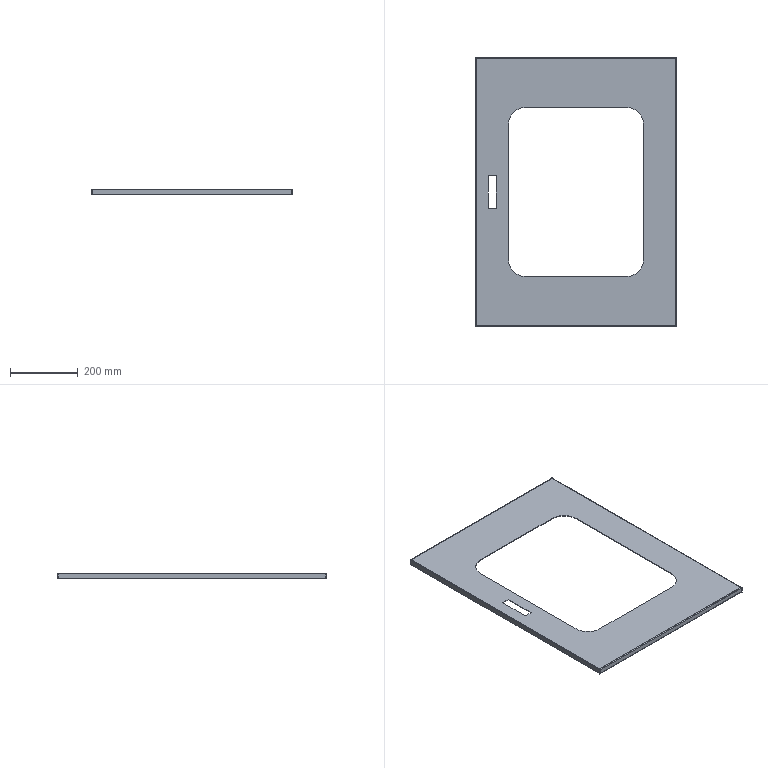Component | SolidWorks | OuterDoor-1 | 1 solid | 148 faces | volume 647702 mm3 | plane 102 | cylinder 42 | spline 4 | commonest cylinder face diameters 3.2 x24 4.2 x7 0.2 x7 100 x4